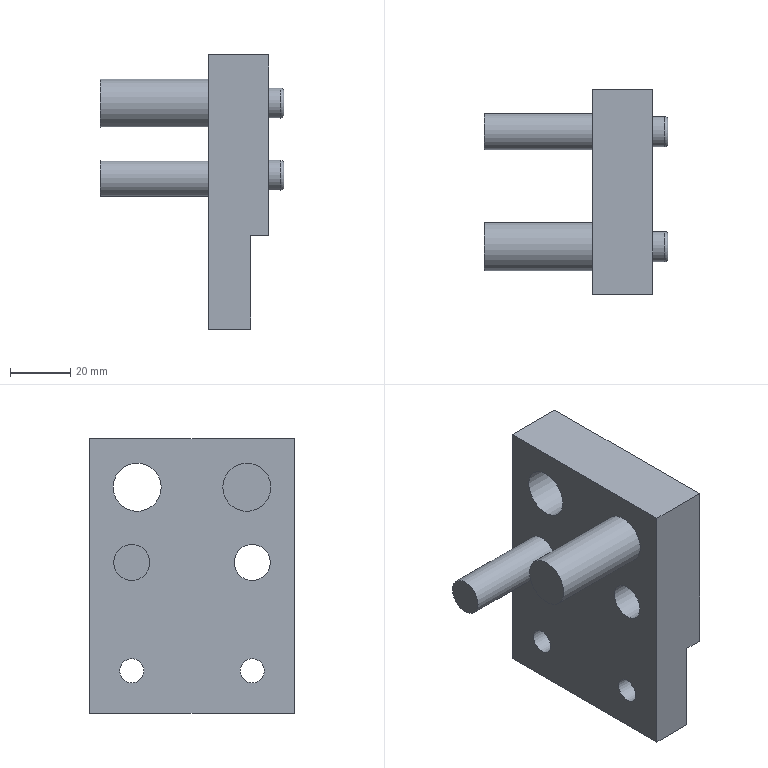Component | NX | CLAMP_CYL_COMP_2 | 1 solid | 38 faces | volume 110423 mm3 | plane 18 | cylinder 14 | torus 4 | cone 2 | commonest cylinder face diameters 16 x4 25 x2 20 x2 8 x2 12 x2 10 x2